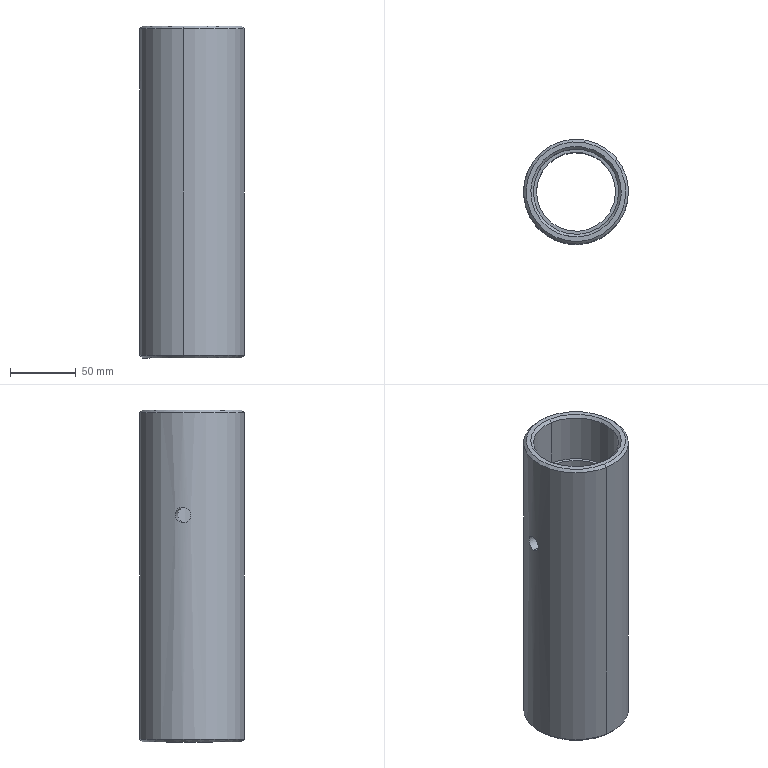Component | SolidWorks | VerticalShaftSleeve-2 | 1 solid | 19 faces | box 80 x 80 x 253 mm | volume 529804 mm3 | cone 8 | cylinder 8 | plane 3 | commonest cylinder face diameters 12 x2 65 x2 80 x2 60.2 x2 | material Q235
build123d program:
from build123d import *

# Parameters (mm, degrees)
SKETCH1_R           = 40
SKETCH1_R_2         = 30.1
BOSS_EXTRUDE1_DEPTH = 253
SKETCH2_R           = 32.5
CUT_EXTRUDE1_DEPTH  = 40
SKETCH3_R           = 6
CUT_EXTRUDE2_DEPTH  = 40
CHAMFER1_SIZE       = 2
CHAMFER2_SIZE       = 2


with BuildPart() as part:
    # Sketch1 → Boss-Extrude1 (new body)
    with BuildSketch(Plane.XY):
        Circle(SKETCH1_R)
        Circle(SKETCH1_R_2, mode=Mode.SUBTRACT)
    extrude(amount=BOSS_EXTRUDE1_DEPTH)

    # Sketch2 → Cut-Extrude1 (cut)
    with BuildSketch(Plane(origin=(0, 0, 0), x_dir=(-1, 0, 0), z_dir=(0, 0, -1))):
        Circle(SKETCH2_R)
    extrude(amount=-CUT_EXTRUDE1_DEPTH, mode=Mode.SUBTRACT)

    # Sketch3 → Cut-Extrude2 (cut)
    with BuildSketch(Plane(origin=(0, 0, 0), x_dir=(1, 0, 0), z_dir=(0, 1, 0))):
        with Locations(Location((0, -80, 0), (0, 0, 270))):
            Circle(SKETCH3_R)
    extrude(amount=-CUT_EXTRUDE2_DEPTH, mode=Mode.SUBTRACT)

    # Chamfer1
    chamfer1_edges = [part.edges().sort_by_distance(p)[0] for p in [
        (-40, 0, 0),
        (-40, 0, 253),
    ]]
    chamfer(chamfer1_edges, length=CHAMFER1_SIZE)

    # Chamfer2
    chamfer2_edges = [part.edges().sort_by_distance(p)[0] for p in [
        (32.5, 0, 0),
        (-30.1, 0, 253),
    ]]
    chamfer(chamfer2_edges, length=CHAMFER2_SIZE)


solid = part.part

# Placed as in the assembly
solid = solid.moved(Location((-277.654, 1601.474, 2931.295), (-180, 0, -80.097)))
STEP:
#1=COLOUR_RGB('',0.7922,0.8196,0.9333);
#2=FILL_AREA_STYLE_COLOUR('',#1);
#3=FILL_AREA_STYLE('',(#2));
#4=SURFACE_STYLE_FILL_AREA(#3);
#5=SURFACE_SIDE_STYLE('',(#4));
#6=SURFACE_STYLE_USAGE(.BOTH.,#5);
#7=PRESENTATION_STYLE_ASSIGNMENT((#6));
#8=CARTESIAN_POINT('',(-10.712,64.311,115.327));
#9=VERTEX_POINT('',#8);
#10=CARTESIAN_POINT('',(-11.151,61.79,115.327));
#11=VERTEX_POINT('',#10);
#12=CARTESIAN_POINT('',(-10.931,63.05,115.327));
#13=DIRECTION('',(-0.,-0.,1.));
#14=DIRECTION('',(0.1718,0.9851,0.));
#15=AXIS2_PLACEMENT_3D('',#12,#13,#14);
#16=CIRCLE('',#15,1.28);
#17=EDGE_CURVE('',#9,#11,#16,.T.);
#18=ORIENTED_EDGE('',*,*,#17,.F.);
#19=CARTESIAN_POINT('',(-10.698,64.388,115.405));
#20=VERTEX_POINT('',#19);
#21=CARTESIAN_POINT('',(-10.712,64.311,115.327));
#22=DIRECTION('',(0.1214,0.6966,0.7071));
#23=VECTOR('',#22,39.37);
#24=LINE('',#21,#23);
#25=EDGE_CURVE('',#9,#20,#24,.T.);
#26=ORIENTED_EDGE('',*,*,#25,.T.);
#27=CARTESIAN_POINT('',(-11.165,61.712,115.405));
#28=VERTEX_POINT('',#27);
#29=CARTESIAN_POINT('',(-10.931,63.05,115.405));
#30=DIRECTION('',(0.,0.,-1.));
#31=DIRECTION('',(0.1718,0.9851,0.));
#32=AXIS2_PLACEMENT_3D('',#29,#30,#31);
#33=CIRCLE('',#32,1.358);
#34=EDGE_CURVE('',#28,#20,#33,.T.);
#35=ORIENTED_EDGE('',*,*,#34,.F.);
#36=CARTESIAN_POINT('',(-11.151,61.79,115.327));
#37=DIRECTION('',(-0.1214,-0.6966,0.7071));
#38=VECTOR('',#37,39.37);
#39=LINE('',#36,#38);
#40=EDGE_CURVE('',#11,#28,#39,.T.);
#41=ORIENTED_EDGE('',*,*,#40,.F.);
#42=EDGE_LOOP('',(#18,#26,#35,#41));
#43=FACE_OUTER_BOUND('',#42,.T.);
#44=CARTESIAN_POINT('',(-10.931,63.05,115.327));
#45=DIRECTION('',(-0.,-0.,1.));
#46=DIRECTION('',(-0.1718,-0.9851,0.));
#47=AXIS2_PLACEMENT_3D('',#44,#45,#46);
#48=CONICAL_SURFACE('',#47,1.28,0.7854);
#49=ADVANCED_FACE('',(#43),#48,.F.);
#50=CARTESIAN_POINT('',(-11.135,61.883,105.523));
#51=VERTEX_POINT('',#50);
#52=CARTESIAN_POINT('',(-10.728,64.218,105.523));
#53=VERTEX_POINT('',#52);
#54=CARTESIAN_POINT('',(-10.931,63.05,105.523));
#55=DIRECTION('',(0.,0.,-1.));
#56=DIRECTION('',(0.1718,0.9851,0.));
#57=AXIS2_PLACEMENT_3D('',#54,#55,#56);
#58=CIRCLE('',#57,1.185);
#59=EDGE_CURVE('',#51,#53,#58,.T.);
#60=ORIENTED_EDGE('',*,*,#59,.F.);
#61=CARTESIAN_POINT('',(-11.148,61.805,105.445));
#62=VERTEX_POINT('',#61);
#63=CARTESIAN_POINT('',(-11.135,61.883,105.523));
#64=DIRECTION('',(-0.1214,-0.6966,-0.7071));
#65=VECTOR('',#64,39.37);
#66=LINE('',#63,#65);
#67=EDGE_CURVE('',#51,#62,#66,.T.);
#68=ORIENTED_EDGE('',*,*,#67,.T.);
#69=CARTESIAN_POINT('',(-10.714,64.295,105.445));
#70=VERTEX_POINT('',#69);
#71=CARTESIAN_POINT('',(-10.931,63.05,105.445));
#72=DIRECTION('',(-0.,-0.,1.));
#73=DIRECTION('',(0.1718,0.9851,0.));
#74=AXIS2_PLACEMENT_3D('',#71,#72,#73);
#75=CIRCLE('',#74,1.264);
#76=EDGE_CURVE('',#70,#62,#75,.T.);
#77=ORIENTED_EDGE('',*,*,#76,.F.);
#78=CARTESIAN_POINT('',(-10.728,64.218,105.523));
#79=DIRECTION('',(0.1214,0.6966,-0.7071));
#80=VECTOR('',#79,39.37);
#81=LINE('',#78,#80);
#82=EDGE_CURVE('',#53,#70,#81,.T.);
#83=ORIENTED_EDGE('',*,*,#82,.F.);
#84=EDGE_LOOP('',(#60,#68,#77,#83));
#85=FACE_OUTER_BOUND('',#84,.T.);
#86=CARTESIAN_POINT('',(-10.931,63.05,105.523));
#87=DIRECTION('',(0.,0.,-1.));
#88=DIRECTION('',(0.1718,0.9851,0.));
#89=AXIS2_PLACEMENT_3D('',#86,#87,#88);
#90=CONICAL_SURFACE('',#89,1.185,0.7854);
#91=ADVANCED_FACE('',(#85),#90,.F.);
#92=CARTESIAN_POINT('',(-11.188,61.576,115.405));
#93=VERTEX_POINT('',#92);
#94=CARTESIAN_POINT('',(-10.674,64.524,115.405));
#95=VERTEX_POINT('',#94);
#96=CARTESIAN_POINT('',(-10.931,63.05,115.405));
#97=DIRECTION('',(-0.,-0.,1.));
#98=DIRECTION('',(0.1718,0.9851,0.));
#99=AXIS2_PLACEMENT_3D('',#96,#97,#98);
#100=CIRCLE('',#99,1.496);
#101=EDGE_CURVE('',#93,#95,#100,.T.);
#102=ORIENTED_EDGE('',*,*,#101,.F.);
#103=CARTESIAN_POINT('',(-11.202,61.499,115.327));
#104=VERTEX_POINT('',#103);
#105=CARTESIAN_POINT('',(-11.202,61.499,115.327));
#106=DIRECTION('',(-0.1214,-0.6966,-0.7071));
#107=VECTOR('',#106,39.37);
#108=LINE('',#105,#107);
#109=EDGE_CURVE('',#93,#104,#108,.T.);
#110=ORIENTED_EDGE('',*,*,#109,.T.);
#111=CARTESIAN_POINT('',(-10.661,64.602,115.327));
#112=VERTEX_POINT('',#111);
#113=CARTESIAN_POINT('',(-10.931,63.05,115.327));
#114=DIRECTION('',(0.,0.,-1.));
#115=DIRECTION('',(0.1718,0.9851,0.));
#116=AXIS2_PLACEMENT_3D('',#113,#114,#115);
#117=CIRCLE('',#116,1.575);
#118=EDGE_CURVE('',#112,#104,#117,.T.);
#119=ORIENTED_EDGE('',*,*,#118,.F.);
#120=CARTESIAN_POINT('',(-10.661,64.602,115.327));
#121=DIRECTION('',(0.1214,0.6966,-0.7071));
#122=VECTOR('',#121,39.37);
#123=LINE('',#120,#122);
#124=EDGE_CURVE('',#95,#112,#123,.T.);
#125=ORIENTED_EDGE('',*,*,#124,.F.);
#126=EDGE_LOOP('',(#102,#110,#119,#125));
#127=FACE_OUTER_BOUND('',#126,.T.);
#128=CARTESIAN_POINT('',(-10.931,63.05,115.327));
#129=DIRECTION('',(0.,0.,-1.));
#130=DIRECTION('',(0.1718,0.9851,0.));
#131=AXIS2_PLACEMENT_3D('',#128,#129,#130);
#132=CONICAL_SURFACE('',#131,1.575,0.7854);
#133=ADVANCED_FACE('',(#127),#132,.T.);
#134=CARTESIAN_POINT('',(-10.674,64.524,105.445));
#135=VERTEX_POINT('',#134);
#136=CARTESIAN_POINT('',(-11.188,61.576,105.445));
#137=VERTEX_POINT('',#136);
#138=CARTESIAN_POINT('',(-10.931,63.05,105.445));
#139=DIRECTION('',(0.,0.,-1.));
#140=DIRECTION('',(0.1718,0.9851,0.));
#141=AXIS2_PLACEMENT_3D('',#138,#139,#140);
#142=CIRCLE('',#141,1.496);
#143=EDGE_CURVE('',#135,#137,#142,.T.);
#144=ORIENTED_EDGE('',*,*,#143,.F.);
#145=CARTESIAN_POINT('',(-10.661,64.602,105.523));
#146=VERTEX_POINT('',#145);
#147=CARTESIAN_POINT('',(-10.674,64.524,105.445));
#148=DIRECTION('',(0.1214,0.6966,0.7071));
#149=VECTOR('',#148,39.37);
#150=LINE('',#147,#149);
#151=EDGE_CURVE('',#135,#146,#150,.T.);
#152=ORIENTED_EDGE('',*,*,#151,.T.);
#153=CARTESIAN_POINT('',(-11.202,61.499,105.523));
#154=VERTEX_POINT('',#153);
#155=CARTESIAN_POINT('',(-10.931,63.05,105.523));
#156=DIRECTION('',(-0.,-0.,1.));
#157=DIRECTION('',(0.1718,0.9851,0.));
#158=AXIS2_PLACEMENT_3D('',#155,#156,#157);
#159=CIRCLE('',#158,1.575);
#160=EDGE_CURVE('',#154,#146,#159,.T.);
#161=ORIENTED_EDGE('',*,*,#160,.F.);
#162=CARTESIAN_POINT('',(-11.188,61.576,105.445));
#163=DIRECTION('',(-0.1214,-0.6966,0.7071));
#164=VECTOR('',#163,39.37);
#165=LINE('',#162,#164);
#166=EDGE_CURVE('',#137,#154,#165,.T.);
#167=ORIENTED_EDGE('',*,*,#166,.F.);
#168=EDGE_LOOP('',(#144,#152,#161,#167));
#169=FACE_OUTER_BOUND('',#168,.T.);
#170=CARTESIAN_POINT('',(-10.931,63.05,105.445));
#171=DIRECTION('',(-0.,-0.,1.));
#172=DIRECTION('',(-0.1718,-0.9851,0.));
#173=AXIS2_PLACEMENT_3D('',#170,#171,#172);
#174=CONICAL_SURFACE('',#173,1.496,0.7854);
#175=ADVANCED_FACE('',(#169),#174,.T.);
#176=CARTESIAN_POINT('',(-12.483,63.321,112.492));
#177=VERTEX_POINT('',#176);
#178=CARTESIAN_POINT('',(-12.483,63.321,112.019));
#179=VERTEX_POINT('',#178);
#180=CARTESIAN_POINT('',(-12.483,63.321,112.492));
#181=CARTESIAN_POINT('',(-12.485,63.305,112.492));
#182=CARTESIAN_POINT('',(-12.488,63.29,112.49));
#183=CARTESIAN_POINT('',(-12.492,63.26,112.484));
#184=CARTESIAN_POINT('',(-12.494,63.245,112.48));
#185=CARTESIAN_POINT('',(-12.496,63.224,112.471));
#186=CARTESIAN_POINT('',(-12.497,63.217,112.468));
#187=CARTESIAN_POINT('',(-12.499,63.204,112.46));
#188=CARTESIAN_POINT('',(-12.499,63.197,112.456));
#189=CARTESIAN_POINT('',(-12.501,63.177,112.443));
#190=CARTESIAN_POINT('',(-12.502,63.166,112.434));
#191=CARTESIAN_POINT('',(-12.503,63.144,112.412));
#192=CARTESIAN_POINT('',(-12.504,63.134,112.4));
#193=CARTESIAN_POINT('',(-12.505,63.116,112.374));
#194=CARTESIAN_POINT('',(-12.505,63.109,112.361));
#195=CARTESIAN_POINT('',(-12.505,63.1,112.339));
#196=CARTESIAN_POINT('',(-12.505,63.097,112.332));
#197=CARTESIAN_POINT('',(-12.505,63.093,112.317));
#198=CARTESIAN_POINT('',(-12.506,63.091,112.31));
#199=CARTESIAN_POINT('',(-12.506,63.086,112.287));
#200=CARTESIAN_POINT('',(-12.506,63.085,112.271));
#201=CARTESIAN_POINT('',(-12.506,63.085,112.24));
#202=CARTESIAN_POINT('',(-12.506,63.086,112.225));
#203=CARTESIAN_POINT('',(-12.506,63.091,112.202));
#204=CARTESIAN_POINT('',(-12.505,63.093,112.195));
#205=CARTESIAN_POINT('',(-12.505,63.097,112.18));
#206=CARTESIAN_POINT('',(-12.505,63.1,112.172));
#207=CARTESIAN_POINT('',(-12.505,63.109,112.151));
#208=CARTESIAN_POINT('',(-12.505,63.116,112.137));
#209=CARTESIAN_POINT('',(-12.504,63.134,112.112));
#210=CARTESIAN_POINT('',(-12.503,63.144,112.1));
#211=CARTESIAN_POINT('',(-12.502,63.165,112.078));
#212=CARTESIAN_POINT('',(-12.501,63.177,112.068));
#213=CARTESIAN_POINT('',(-12.499,63.203,112.051));
#214=CARTESIAN_POINT('',(-12.497,63.217,112.044));
#215=CARTESIAN_POINT('',(-12.495,63.238,112.035));
#216=CARTESIAN_POINT('',(-12.494,63.245,112.032));
#217=CARTESIAN_POINT('',(-12.492,63.26,112.028));
#218=CARTESIAN_POINT('',(-12.491,63.267,112.026));
#219=CARTESIAN_POINT('',(-12.488,63.29,112.021));
#220=CARTESIAN_POINT('',(-12.485,63.305,112.019));
#221=CARTESIAN_POINT('',(-12.483,63.321,112.019));
#222=B_SPLINE_CURVE_WITH_KNOTS('',3,(#180,#181,#182,#183,#184,#185,#186,#187,#188,#189,#190,#191,#192,#193,#194,#195,#196,#197,#198,#199,#200,#201,#202,#203,#204,#205,#206,#207,#208,#209,#210,#211,#212,#213,#214,#215,#216,#217,#218,#219,#220,#221),.UNSPECIFIED.,.F.,.F.,(4,2,2,2,2,2,2,2,2,2,2,2,2,2,2,2,2,2,2,2,4),(0.01879,0.01996,0.02113,0.02172,0.02231,0.02348,0.02465,0.02583,0.02641,0.027,0.02818,0.02935,0.02994,0.03052,0.0317,0.03287,0.03404,0.03522,0.03581,0.03639,0.03757),.UNSPECIFIED.);
#223=EDGE_CURVE('',#177,#179,#222,.T.);
#224=ORIENTED_EDGE('',*,*,#223,.F.);
#225=CARTESIAN_POINT('',(-12.099,63.254,112.492));
#226=VERTEX_POINT('',#225);
#227=CARTESIAN_POINT('',(-12.483,63.321,112.492));
#228=DIRECTION('',(0.9851,-0.1718,0.));
#229=VECTOR('',#228,39.37);
#230=LINE('',#227,#229);
#231=EDGE_CURVE('',#177,#226,#230,.T.);
#232=ORIENTED_EDGE('',*,*,#231,.T.);
#233=CARTESIAN_POINT('',(-12.099,63.254,112.019));
#234=VERTEX_POINT('',#233);
#235=CARTESIAN_POINT('',(-12.099,63.254,112.492));
#236=CARTESIAN_POINT('',(-12.101,63.238,112.492));
#237=CARTESIAN_POINT('',(-12.104,63.223,112.49));
#238=CARTESIAN_POINT('',(-12.108,63.193,112.484));
#239=CARTESIAN_POINT('',(-12.109,63.178,112.48));
#240=CARTESIAN_POINT('',(-12.112,63.157,112.471));
#241=CARTESIAN_POINT('',(-12.112,63.15,112.468));
#242=CARTESIAN_POINT('',(-12.113,63.136,112.46));
#243=CARTESIAN_POINT('',(-12.114,63.13,112.456));
#244=CARTESIAN_POINT('',(-12.115,63.11,112.443));
#245=CARTESIAN_POINT('',(-12.115,63.098,112.434));
#246=CARTESIAN_POINT('',(-12.116,63.076,112.412));
#247=CARTESIAN_POINT('',(-12.116,63.066,112.4));
#248=CARTESIAN_POINT('',(-12.116,63.049,112.374));
#249=CARTESIAN_POINT('',(-12.116,63.041,112.361));
#250=CARTESIAN_POINT('',(-12.116,63.032,112.339));
#251=CARTESIAN_POINT('',(-12.116,63.03,112.332));
#252=CARTESIAN_POINT('',(-12.116,63.025,112.317));
#253=CARTESIAN_POINT('',(-12.116,63.023,112.31));
#254=CARTESIAN_POINT('',(-12.116,63.018,112.287));
#255=CARTESIAN_POINT('',(-12.116,63.017,112.271));
#256=CARTESIAN_POINT('',(-12.116,63.017,112.24));
#257=CARTESIAN_POINT('',(-12.116,63.018,112.225));
#258=CARTESIAN_POINT('',(-12.116,63.025,112.195));
#259=CARTESIAN_POINT('',(-12.116,63.029,112.18));
#260=CARTESIAN_POINT('',(-12.116,63.041,112.151));
#261=CARTESIAN_POINT('',(-12.116,63.049,112.137));
#262=CARTESIAN_POINT('',(-12.116,63.062,112.118));
#263=CARTESIAN_POINT('',(-12.116,63.066,112.112));
#264=CARTESIAN_POINT('',(-12.116,63.076,112.1));
#265=CARTESIAN_POINT('',(-12.116,63.082,112.094));
#266=CARTESIAN_POINT('',(-12.115,63.098,112.078));
#267=CARTESIAN_POINT('',(-12.115,63.11,112.068));
#268=CARTESIAN_POINT('',(-12.113,63.136,112.051));
#269=CARTESIAN_POINT('',(-12.112,63.15,112.044));
#270=CARTESIAN_POINT('',(-12.11,63.171,112.035));
#271=CARTESIAN_POINT('',(-12.109,63.178,112.032));
#272=CARTESIAN_POINT('',(-12.108,63.193,112.028));
#273=CARTESIAN_POINT('',(-12.107,63.2,112.026));
#274=CARTESIAN_POINT('',(-12.104,63.223,112.021));
#275=CARTESIAN_POINT('',(-12.101,63.238,112.019));
#276=CARTESIAN_POINT('',(-12.099,63.254,112.019));
#277=B_SPLINE_CURVE_WITH_KNOTS('',3,(#235,#236,#237,#238,#239,#240,#241,#242,#243,#244,#245,#246,#247,#248,#249,#250,#251,#252,#253,#254,#255,#256,#257,#258,#259,#260,#261,#262,#263,#264,#265,#266,#267,#268,#269,#270,#271,#272,#273,#274,#275,#276),.UNSPECIFIED.,.F.,.F.,(4,2,2,2,2,2,2,2,2,2,2,2,2,2,2,2,2,2,2,2,4),(0.01881,0.01998,0.02116,0.02174,0.02233,0.02351,0.02468,0.02586,0.02644,0.02703,0.02821,0.02938,0.03056,0.03173,0.03232,0.03291,0.03408,0.03526,0.03584,0.03643,0.03761),.UNSPECIFIED.);
#278=EDGE_CURVE('',#226,#234,#277,.T.);
#279=ORIENTED_EDGE('',*,*,#278,.T.);
#280=CARTESIAN_POINT('',(-12.483,63.321,112.019));
#281=DIRECTION('',(0.9851,-0.1718,0.));
#282=VECTOR('',#281,39.37);
#283=LINE('',#280,#282);
#284=EDGE_CURVE('',#179,#234,#283,.T.);
#285=ORIENTED_EDGE('',*,*,#284,.F.);
#286=EDGE_LOOP('',(#224,#232,#279,#285));
#287=FACE_OUTER_BOUND('',#286,.T.);
#288=CARTESIAN_POINT('',(-12.483,63.321,112.256));
#289=DIRECTION('',(0.9851,-0.1718,0.));
#290=DIRECTION('',(0.,0.,-1.));
#291=AXIS2_PLACEMENT_3D('',#288,#289,#290);
#292=CYLINDRICAL_SURFACE('',#291,0.2362);
#293=ADVANCED_FACE('',(#287),#292,.F.);
#294=CARTESIAN_POINT('',(-10.712,64.311,113.831));
#295=VERTEX_POINT('',#294);
#296=CARTESIAN_POINT('',(-11.151,61.79,113.831));
#297=VERTEX_POINT('',#296);
#298=CARTESIAN_POINT('',(-10.931,63.05,113.831));
#299=DIRECTION('',(-0.,-0.,1.));
#300=DIRECTION('',(-0.1718,-0.9851,0.));
#301=AXIS2_PLACEMENT_3D('',#298,#299,#300);
#302=CIRCLE('',#301,1.28);
#303=EDGE_CURVE('',#295,#297,#302,.T.);
#304=ORIENTED_EDGE('',*,*,#303,.F.);
#305=CARTESIAN_POINT('',(-10.712,64.311,113.831));
#306=DIRECTION('',(-0.,-0.,1.));
#307=VECTOR('',#306,39.37);
#308=LINE('',#305,#307);
#309=EDGE_CURVE('',#295,#9,#308,.T.);
#310=ORIENTED_EDGE('',*,*,#309,.T.);
#311=ORIENTED_EDGE('',*,*,#17,.T.);
#312=CARTESIAN_POINT('',(-11.151,61.79,113.831));
#313=DIRECTION('',(-0.,-0.,1.));
#314=VECTOR('',#313,39.37);
#315=LINE('',#312,#314);
#316=EDGE_CURVE('',#297,#11,#315,.T.);
#317=ORIENTED_EDGE('',*,*,#316,.F.);
#318=EDGE_LOOP('',(#304,#310,#311,#317));
#319=FACE_OUTER_BOUND('',#318,.T.);
#320=CARTESIAN_POINT('',(-10.931,63.05,113.831));
#321=DIRECTION('',(-0.,-0.,1.));
#322=DIRECTION('',(-0.1718,-0.9851,0.));
#323=AXIS2_PLACEMENT_3D('',#320,#321,#322);
#324=CYLINDRICAL_SURFACE('',#323,1.28);
#325=ADVANCED_FACE('',(#319),#324,.F.);
#326=ORIENTED_EDGE('',*,*,#160,.T.);
#327=CARTESIAN_POINT('',(-10.661,64.602,105.445));
#328=DIRECTION('',(-0.,-0.,1.));
#329=VECTOR('',#328,39.37);
#330=LINE('',#327,#329);
#331=EDGE_CURVE('',#146,#112,#330,.T.);
#332=ORIENTED_EDGE('',*,*,#331,.T.);
#333=ORIENTED_EDGE('',*,*,#118,.T.);
#334=CARTESIAN_POINT('',(-11.202,61.499,105.445));
#335=DIRECTION('',(-0.,-0.,1.));
#336=VECTOR('',#335,39.37);
#337=LINE('',#334,#336);
#338=EDGE_CURVE('',#154,#104,#337,.T.);
#339=ORIENTED_EDGE('',*,*,#338,.F.);
#340=EDGE_LOOP('',(#326,#332,#333,#339));
#341=FACE_OUTER_BOUND('',#340,.T.);
#342=CARTESIAN_POINT('',(-10.931,63.05,105.445));
#343=DIRECTION('',(-0.,-0.,1.));
#344=DIRECTION('',(-0.1718,-0.9851,0.));
#345=AXIS2_PLACEMENT_3D('',#342,#343,#344);
#346=CYLINDRICAL_SURFACE('',#345,1.575);
#347=ADVANCED_FACE('',(#341),#346,.T.);
#348=CARTESIAN_POINT('',(-12.099,63.254,112.019));
#349=CARTESIAN_POINT('',(-12.096,63.269,112.019));
#350=CARTESIAN_POINT('',(-12.093,63.284,112.021));
#351=CARTESIAN_POINT('',(-12.088,63.306,112.026));
#352=CARTESIAN_POINT('',(-12.087,63.314,112.027));
#353=CARTESIAN_POINT('',(-12.083,63.328,112.032));
#354=CARTESIAN_POINT('',(-12.081,63.335,112.035));
#355=CARTESIAN_POINT('',(-12.076,63.356,112.043));
#356=CARTESIAN_POINT('',(-12.073,63.369,112.051));
#357=CARTESIAN_POINT('',(-12.065,63.394,112.068));
#358=CARTESIAN_POINT('',(-12.062,63.406,112.078));
#359=CARTESIAN_POINT('',(-12.055,63.427,112.1));
#360=CARTESIAN_POINT('',(-12.052,63.436,112.111));
#361=CARTESIAN_POINT('',(-12.046,63.453,112.137));
#362=CARTESIAN_POINT('',(-12.043,63.46,112.151));
#363=CARTESIAN_POINT('',(-12.04,63.468,112.172));
#364=CARTESIAN_POINT('',(-12.039,63.47,112.18));
#365=CARTESIAN_POINT('',(-12.038,63.475,112.194));
#366=CARTESIAN_POINT('',(-12.037,63.477,112.202));
#367=CARTESIAN_POINT('',(-12.035,63.481,112.225));
#368=CARTESIAN_POINT('',(-12.035,63.482,112.24));
#369=CARTESIAN_POINT('',(-12.035,63.482,112.271));
#370=CARTESIAN_POINT('',(-12.035,63.481,112.287));
#371=CARTESIAN_POINT('',(-12.038,63.475,112.317));
#372=CARTESIAN_POINT('',(-12.039,63.471,112.332));
#373=CARTESIAN_POINT('',(-12.042,63.462,112.353));
#374=CARTESIAN_POINT('',(-12.043,63.459,112.36));
#375=CARTESIAN_POINT('',(-12.046,63.452,112.374));
#376=CARTESIAN_POINT('',(-12.047,63.448,112.381));
#377=CARTESIAN_POINT('',(-12.052,63.436,112.4));
#378=CARTESIAN_POINT('',(-12.055,63.427,112.412));
#379=CARTESIAN_POINT('',(-12.062,63.406,112.434));
#380=CARTESIAN_POINT('',(-12.065,63.394,112.443));
#381=CARTESIAN_POINT('',(-12.071,63.376,112.456));
#382=CARTESIAN_POINT('',(-12.073,63.369,112.46));
#383=CARTESIAN_POINT('',(-12.076,63.356,112.468));
#384=CARTESIAN_POINT('',(-12.078,63.349,112.471));
#385=CARTESIAN_POINT('',(-12.083,63.328,112.48));
#386=CARTESIAN_POINT('',(-12.087,63.314,112.484));
#387=CARTESIAN_POINT('',(-12.091,63.292,112.489));
#388=CARTESIAN_POINT('',(-12.093,63.284,112.49));
#389=CARTESIAN_POINT('',(-12.096,63.269,112.492));
#390=CARTESIAN_POINT('',(-12.097,63.261,112.492));
#391=CARTESIAN_POINT('',(-12.099,63.254,112.492));
#392=B_SPLINE_CURVE_WITH_KNOTS('',3,(#348,#349,#350,#351,#352,#353,#354,#355,#356,#357,#358,#359,#360,#361,#362,#363,#364,#365,#366,#367,#368,#369,#370,#371,#372,#373,#374,#375,#376,#377,#378,#379,#380,#381,#382,#383,#384,#385,#386,#387,#388,#389,#390,#391),.UNSPECIFIED.,.F.,.F.,(4,2,2,2,2,2,2,2,2,2,2,2,2,2,2,2,2,2,2,2,2,4),(0.,0.001175,0.001763,0.002351,0.003526,0.004701,0.005877,0.007052,0.00764,0.008228,0.009403,0.01058,0.01175,0.01234,0.01293,0.0141,0.01528,0.01587,0.01646,0.01763,0.01822,0.01881),.UNSPECIFIED.);
#393=EDGE_CURVE('',#234,#226,#392,.T.);
#394=ORIENTED_EDGE('',*,*,#393,.F.);
#395=ORIENTED_EDGE('',*,*,#278,.F.);
#396=EDGE_LOOP('',(#394,#395));
#397=FACE_BOUND('',#396,.T.);
#398=ORIENTED_EDGE('',*,*,#59,.T.);
#399=CARTESIAN_POINT('',(-10.728,64.218,113.831));
#400=VERTEX_POINT('',#399);
#401=CARTESIAN_POINT('',(-10.728,64.218,105.445));
#402=DIRECTION('',(-0.,-0.,1.));
#403=VECTOR('',#402,39.37);
#404=LINE('',#401,#403);
#405=EDGE_CURVE('',#53,#400,#404,.T.);
#406=ORIENTED_EDGE('',*,*,#405,.T.);
#407=CARTESIAN_POINT('',(-11.135,61.883,113.831));
#408=VERTEX_POINT('',#407);
#409=CARTESIAN_POINT('',(-10.931,63.05,113.831));
#410=DIRECTION('',(-0.,-0.,1.));
#411=DIRECTION('',(-0.1718,-0.9851,0.));
#412=AXIS2_PLACEMENT_3D('',#409,#410,#411);
#413=CIRCLE('',#412,1.185);
#414=EDGE_CURVE('',#400,#408,#413,.T.);
#415=ORIENTED_EDGE('',*,*,#414,.T.);
#416=CARTESIAN_POINT('',(-11.135,61.883,105.445));
#417=DIRECTION('',(-0.,-0.,1.));
#418=VECTOR('',#417,39.37);
#419=LINE('',#416,#418);
#420=EDGE_CURVE('',#51,#408,#419,.T.);
#421=ORIENTED_EDGE('',*,*,#420,.F.);
#422=EDGE_LOOP('',(#398,#406,#415,#421));
#423=FACE_OUTER_BOUND('',#422,.T.);
#424=CARTESIAN_POINT('',(-10.931,63.05,105.445));
#425=DIRECTION('',(-0.,-0.,1.));
#426=DIRECTION('',(-0.1718,-0.9851,0.));
#427=AXIS2_PLACEMENT_3D('',#424,#425,#426);
#428=CYLINDRICAL_SURFACE('',#427,1.185);
#429=ADVANCED_FACE('',(#397,#423),#428,.F.);
#430=ORIENTED_EDGE('',*,*,#405,.F.);
#431=CARTESIAN_POINT('',(-10.931,63.05,105.523));
#432=DIRECTION('',(0.,0.,-1.));
#433=DIRECTION('',(0.1718,0.9851,0.));
#434=AXIS2_PLACEMENT_3D('',#431,#432,#433);
#435=CIRCLE('',#434,1.185);
#436=EDGE_CURVE('',#53,#51,#435,.T.);
#437=ORIENTED_EDGE('',*,*,#436,.T.);
#438=ORIENTED_EDGE('',*,*,#420,.T.);
#439=CARTESIAN_POINT('',(-10.931,63.05,113.831));
#440=DIRECTION('',(-0.,-0.,1.));
#441=DIRECTION('',(-0.1718,-0.9851,0.));
#442=AXIS2_PLACEMENT_3D('',#439,#440,#441);
#443=CIRCLE('',#442,1.185);
#444=EDGE_CURVE('',#408,#400,#443,.T.);
#445=ORIENTED_EDGE('',*,*,#444,.T.);
#446=EDGE_LOOP('',(#430,#437,#438,#445));
#447=FACE_OUTER_BOUND('',#446,.T.);
#448=CARTESIAN_POINT('',(-10.931,63.05,105.445));
#449=DIRECTION('',(-0.,-0.,1.));
#450=DIRECTION('',(-0.1718,-0.9851,0.));
#451=AXIS2_PLACEMENT_3D('',#448,#449,#450);
#452=CYLINDRICAL_SURFACE('',#451,1.185);
#453=ADVANCED_FACE('',(#447),#452,.F.);
#454=ORIENTED_EDGE('',*,*,#76,.T.);
#455=CARTESIAN_POINT('',(-10.931,63.05,105.445));
#456=DIRECTION('',(-0.,-0.,1.));
#457=DIRECTION('',(0.1718,0.9851,0.));
#458=AXIS2_PLACEMENT_3D('',#455,#456,#457);
#459=CIRCLE('',#458,1.264);
#460=EDGE_CURVE('',#62,#70,#459,.T.);
#461=ORIENTED_EDGE('',*,*,#460,.T.);
#462=EDGE_LOOP('',(#454,#461));
#463=FACE_BOUND('',#462,.T.);
#464=CARTESIAN_POINT('',(-10.931,63.05,105.445));
#465=DIRECTION('',(0.,0.,-1.));
#466=DIRECTION('',(0.1718,0.9851,0.));
#467=AXIS2_PLACEMENT_3D('',#464,#465,#466);
#468=CIRCLE('',#467,1.496);
#469=EDGE_CURVE('',#137,#135,#468,.T.);
#470=ORIENTED_EDGE('',*,*,#469,.T.);
#471=ORIENTED_EDGE('',*,*,#143,.T.);
#472=EDGE_LOOP('',(#470,#471));
#473=FACE_OUTER_BOUND('',#472,.T.);
#474=CARTESIAN_POINT('',(-10.931,63.05,105.445));
#475=DIRECTION('',(0.,0.,-1.));
#476=DIRECTION('',(0.1718,0.9851,0.));
#477=AXIS2_PLACEMENT_3D('',#474,#475,#476);
#478=PLANE('',#477);
#479=ADVANCED_FACE('',(#463,#473),#478,.T.);
#480=ORIENTED_EDGE('',*,*,#34,.T.);
#481=CARTESIAN_POINT('',(-10.931,63.05,115.405));
#482=DIRECTION('',(0.,0.,-1.));
#483=DIRECTION('',(0.1718,0.9851,0.));
#484=AXIS2_PLACEMENT_3D('',#481,#482,#483);
#485=CIRCLE('',#484,1.358);
#486=EDGE_CURVE('',#20,#28,#485,.T.);
#487=ORIENTED_EDGE('',*,*,#486,.T.);
#488=EDGE_LOOP('',(#480,#487));
#489=FACE_BOUND('',#488,.T.);
#490=CARTESIAN_POINT('',(-10.931,63.05,115.405));
#491=DIRECTION('',(-0.,-0.,1.));
#492=DIRECTION('',(0.1718,0.9851,0.));
#493=AXIS2_PLACEMENT_3D('',#490,#491,#492);
#494=CIRCLE('',#493,1.496);
#495=EDGE_CURVE('',#95,#93,#494,.T.);
#496=ORIENTED_EDGE('',*,*,#495,.T.);
#497=ORIENTED_EDGE('',*,*,#101,.T.);
#498=EDGE_LOOP('',(#496,#497));
#499=FACE_OUTER_BOUND('',#498,.T.);
#500=CARTESIAN_POINT('',(-10.931,63.05,115.405));
#501=DIRECTION('',(0.,0.,-1.));
#502=DIRECTION('',(0.1718,0.9851,0.));
#503=AXIS2_PLACEMENT_3D('',#500,#501,#502);
#504=PLANE('',#503);
#505=ADVANCED_FACE('',(#489,#499),#504,.F.);
#506=ORIENTED_EDGE('',*,*,#331,.F.);
#507=CARTESIAN_POINT('',(-10.931,63.05,105.523));
#508=DIRECTION('',(-0.,-0.,1.));
#509=DIRECTION('',(0.1718,0.9851,0.));
#510=AXIS2_PLACEMENT_3D('',#507,#508,#509);
#511=CIRCLE('',#510,1.575);
#512=EDGE_CURVE('',#146,#154,#511,.T.);
#513=ORIENTED_EDGE('',*,*,#512,.T.);
#514=ORIENTED_EDGE('',*,*,#338,.T.);
#515=CARTESIAN_POINT('',(-10.931,63.05,115.327));
#516=DIRECTION('',(0.,0.,-1.));
#517=DIRECTION('',(0.1718,0.9851,0.));
#518=AXIS2_PLACEMENT_3D('',#515,#516,#517);
#519=CIRCLE('',#518,1.575);
#520=EDGE_CURVE('',#104,#112,#519,.T.);
#521=ORIENTED_EDGE('',*,*,#520,.T.);
#522=EDGE_LOOP('',(#506,#513,#514,#521));
#523=FACE_OUTER_BOUND('',#522,.T.);
#524=CARTESIAN_POINT('',(-12.483,63.321,112.019));
#525=CARTESIAN_POINT('',(-12.48,63.336,112.019));
#526=CARTESIAN_POINT('',(-12.477,63.351,112.021));
#527=CARTESIAN_POINT('',(-12.473,63.373,112.026));
#528=CARTESIAN_POINT('',(-12.471,63.381,112.027));
#529=CARTESIAN_POINT('',(-12.468,63.395,112.032));
#530=CARTESIAN_POINT('',(-12.466,63.402,112.035));
#531=CARTESIAN_POINT('',(-12.461,63.423,112.043));
#532=CARTESIAN_POINT('',(-12.458,63.437,112.051));
#533=CARTESIAN_POINT('',(-12.451,63.461,112.068));
#534=CARTESIAN_POINT('',(-12.448,63.473,112.078));
#535=CARTESIAN_POINT('',(-12.442,63.494,112.1));
#536=CARTESIAN_POINT('',(-12.439,63.504,112.111));
#537=CARTESIAN_POINT('',(-12.436,63.516,112.131));
#538=CARTESIAN_POINT('',(-12.434,63.52,112.138));
#539=CARTESIAN_POINT('',(-12.432,63.527,112.151));
#540=CARTESIAN_POINT('',(-12.43,63.533,112.165));
#541=CARTESIAN_POINT('',(-12.429,63.538,112.18));
#542=CARTESIAN_POINT('',(-12.427,63.543,112.194));
#543=CARTESIAN_POINT('',(-12.426,63.544,112.202));
#544=CARTESIAN_POINT('',(-12.425,63.549,112.225));
#545=CARTESIAN_POINT('',(-12.425,63.55,112.24));
#546=CARTESIAN_POINT('',(-12.425,63.55,112.271));
#547=CARTESIAN_POINT('',(-12.425,63.549,112.287));
#548=CARTESIAN_POINT('',(-12.427,63.543,112.317));
#549=CARTESIAN_POINT('',(-12.428,63.539,112.332));
#550=CARTESIAN_POINT('',(-12.431,63.53,112.353));
#551=CARTESIAN_POINT('',(-12.432,63.527,112.36));
#552=CARTESIAN_POINT('',(-12.434,63.52,112.374));
#553=CARTESIAN_POINT('',(-12.436,63.516,112.381));
#554=CARTESIAN_POINT('',(-12.439,63.504,112.4));
#555=CARTESIAN_POINT('',(-12.442,63.494,112.412));
#556=CARTESIAN_POINT('',(-12.448,63.473,112.434));
#557=CARTESIAN_POINT('',(-12.451,63.461,112.443));
#558=CARTESIAN_POINT('',(-12.456,63.443,112.456));
#559=CARTESIAN_POINT('',(-12.458,63.436,112.46));
#560=CARTESIAN_POINT('',(-12.461,63.423,112.468));
#561=CARTESIAN_POINT('',(-12.463,63.416,112.471));
#562=CARTESIAN_POINT('',(-12.468,63.395,112.48));
#563=CARTESIAN_POINT('',(-12.471,63.381,112.484));
#564=CARTESIAN_POINT('',(-12.477,63.351,112.49));
#565=CARTESIAN_POINT('',(-12.48,63.336,112.492));
#566=CARTESIAN_POINT('',(-12.483,63.321,112.492));
#567=B_SPLINE_CURVE_WITH_KNOTS('',3,(#524,#525,#526,#527,#528,#529,#530,#531,#532,#533,#534,#535,#536,#537,#538,#539,#540,#541,#542,#543,#544,#545,#546,#547,#548,#549,#550,#551,#552,#553,#554,#555,#556,#557,#558,#559,#560,#561,#562,#563,#564,#565,#566),.UNSPECIFIED.,.F.,.F.,(4,2,2,2,2,2,2,2,1,2,2,2,2,2,2,2,2,2,2,2,2,4),(0.,0.001174,0.001761,0.002348,0.003522,0.004696,0.00587,0.006457,0.007044,0.007632,0.008219,0.009393,0.01057,0.01174,0.01233,0.01291,0.01409,0.01526,0.01585,0.01644,0.01761,0.01879),.UNSPECIFIED.);
#568=EDGE_CURVE('',#179,#177,#567,.T.);
#569=ORIENTED_EDGE('',*,*,#568,.T.);
#570=ORIENTED_EDGE('',*,*,#223,.T.);
#571=EDGE_LOOP('',(#569,#570));
#572=FACE_BOUND('',#571,.T.);
#573=CARTESIAN_POINT('',(-10.931,63.05,105.445));
#574=DIRECTION('',(-0.,-0.,1.));
#575=DIRECTION('',(-0.1718,-0.9851,0.));
#576=AXIS2_PLACEMENT_3D('',#573,#574,#575);
#577=CYLINDRICAL_SURFACE('',#576,1.575);
#578=ADVANCED_FACE('',(#523,#572),#577,.T.);
#579=ORIENTED_EDGE('',*,*,#309,.F.);
#580=CARTESIAN_POINT('',(-10.931,63.05,113.831));
#581=DIRECTION('',(-0.,-0.,1.));
#582=DIRECTION('',(-0.1718,-0.9851,0.));
#583=AXIS2_PLACEMENT_3D('',#580,#581,#582);
#584=CIRCLE('',#583,1.28);
#585=EDGE_CURVE('',#297,#295,#584,.T.);
#586=ORIENTED_EDGE('',*,*,#585,.F.);
#587=ORIENTED_EDGE('',*,*,#316,.T.);
#588=CARTESIAN_POINT('',(-10.931,63.05,115.327));
#589=DIRECTION('',(-0.,-0.,1.));
#590=DIRECTION('',(0.1718,0.9851,0.));
#591=AXIS2_PLACEMENT_3D('',#588,#589,#590);
#592=CIRCLE('',#591,1.28);
#593=EDGE_CURVE('',#11,#9,#592,.T.);
#594=ORIENTED_EDGE('',*,*,#593,.T.);
#595=EDGE_LOOP('',(#579,#586,#587,#594));
#596=FACE_OUTER_BOUND('',#595,.T.);
#597=CARTESIAN_POINT('',(-10.931,63.05,113.831));
#598=DIRECTION('',(-0.,-0.,1.));
#599=DIRECTION('',(-0.1718,-0.9851,0.));
#600=AXIS2_PLACEMENT_3D('',#597,#598,#599);
#601=CYLINDRICAL_SURFACE('',#600,1.28);
#602=ADVANCED_FACE('',(#596),#601,.F.);
#603=ORIENTED_EDGE('',*,*,#444,.F.);
#604=ORIENTED_EDGE('',*,*,#414,.F.);
#605=EDGE_LOOP('',(#603,#604));
#606=FACE_BOUND('',#605,.T.);
#607=ORIENTED_EDGE('',*,*,#585,.T.);
#608=ORIENTED_EDGE('',*,*,#303,.T.);
#609=EDGE_LOOP('',(#607,#608));
#610=FACE_OUTER_BOUND('',#609,.T.);
#611=CARTESIAN_POINT('',(-10.931,63.05,113.831));
#612=DIRECTION('',(-0.,-0.,1.));
#613=DIRECTION('',(-0.1718,-0.9851,-0.));
#614=AXIS2_PLACEMENT_3D('',#611,#612,#613);
#615=PLANE('',#614);
#616=ADVANCED_FACE('',(#606,#610),#615,.T.);
#617=ORIENTED_EDGE('',*,*,#231,.F.);
#618=ORIENTED_EDGE('',*,*,#568,.F.);
#619=ORIENTED_EDGE('',*,*,#284,.T.);
#620=ORIENTED_EDGE('',*,*,#393,.T.);
#621=EDGE_LOOP('',(#617,#618,#619,#620));
#622=FACE_OUTER_BOUND('',#621,.T.);
#623=CARTESIAN_POINT('',(-12.483,63.321,112.256));
#624=DIRECTION('',(0.9851,-0.1718,0.));
#625=DIRECTION('',(0.,0.,-1.));
#626=AXIS2_PLACEMENT_3D('',#623,#624,#625);
#627=CYLINDRICAL_SURFACE('',#626,0.2362);
#628=ADVANCED_FACE('',(#622),#627,.F.);
#629=ORIENTED_EDGE('',*,*,#151,.F.);
#630=ORIENTED_EDGE('',*,*,#469,.F.);
#631=ORIENTED_EDGE('',*,*,#166,.T.);
#632=ORIENTED_EDGE('',*,*,#512,.F.);
#633=EDGE_LOOP('',(#629,#630,#631,#632));
#634=FACE_OUTER_BOUND('',#633,.T.);
#635=CARTESIAN_POINT('',(-10.931,63.05,105.445));
#636=DIRECTION('',(-0.,-0.,1.));
#637=DIRECTION('',(-0.1718,-0.9851,0.));
#638=AXIS2_PLACEMENT_3D('',#635,#636,#637);
#639=CONICAL_SURFACE('',#638,1.496,0.7854);
#640=ADVANCED_FACE('',(#634),#639,.T.);
#641=ORIENTED_EDGE('',*,*,#109,.F.);
#642=ORIENTED_EDGE('',*,*,#495,.F.);
#643=ORIENTED_EDGE('',*,*,#124,.T.);
#644=ORIENTED_EDGE('',*,*,#520,.F.);
#645=EDGE_LOOP('',(#641,#642,#643,#644));
#646=FACE_OUTER_BOUND('',#645,.T.);
#647=CARTESIAN_POINT('',(-10.931,63.05,115.327));
#648=DIRECTION('',(0.,0.,-1.));
#649=DIRECTION('',(0.1718,0.9851,0.));
#650=AXIS2_PLACEMENT_3D('',#647,#648,#649);
#651=CONICAL_SURFACE('',#650,1.575,0.7854);
#652=ADVANCED_FACE('',(#646),#651,.T.);
#653=ORIENTED_EDGE('',*,*,#67,.F.);
#654=ORIENTED_EDGE('',*,*,#436,.F.);
#655=ORIENTED_EDGE('',*,*,#82,.T.);
#656=ORIENTED_EDGE('',*,*,#460,.F.);
#657=EDGE_LOOP('',(#653,#654,#655,#656));
#658=FACE_OUTER_BOUND('',#657,.T.);
#659=CARTESIAN_POINT('',(-10.931,63.05,105.523));
#660=DIRECTION('',(0.,0.,-1.));
#661=DIRECTION('',(0.1718,0.9851,0.));
#662=AXIS2_PLACEMENT_3D('',#659,#660,#661);
#663=CONICAL_SURFACE('',#662,1.185,0.7854);
#664=ADVANCED_FACE('',(#658),#663,.F.);
#665=ORIENTED_EDGE('',*,*,#25,.F.);
#666=ORIENTED_EDGE('',*,*,#593,.F.);
#667=ORIENTED_EDGE('',*,*,#40,.T.);
#668=ORIENTED_EDGE('',*,*,#486,.F.);
#669=EDGE_LOOP('',(#665,#666,#667,#668));
#670=FACE_OUTER_BOUND('',#669,.T.);
#671=CARTESIAN_POINT('',(-10.931,63.05,115.327));
#672=DIRECTION('',(-0.,-0.,1.));
#673=DIRECTION('',(-0.1718,-0.9851,0.));
#674=AXIS2_PLACEMENT_3D('',#671,#672,#673);
#675=CONICAL_SURFACE('',#674,1.28,0.7854);
#676=ADVANCED_FACE('',(#670),#675,.F.);
#677=CLOSED_SHELL('',(#49,#91,#133,#175,#293,#325,#347,#429,#453,#479,#505,#578,#602,#616,#628,#640,#652,#664,#676));
#678=MANIFOLD_SOLID_BREP('',#677);
#679=STYLED_ITEM('',(#7),#678);
#680=PRESENTATION_LAYER_ASSIGNMENT('','',(#679));
#681=CARTESIAN_POINT('',(0.,0.,0.));
#682=DIRECTION('',(0.,0.,1.));
#683=DIRECTION('',(1.,0.,0.));
#684=AXIS2_PLACEMENT_3D('',#681,#682,#683);
#685=(LENGTH_UNIT()NAMED_UNIT(*)SI_UNIT($,.METRE.));
#686=LENGTH_MEASURE_WITH_UNIT(LENGTH_MEASURE(0.0254),#685);
#687=DIMENSIONAL_EXPONENTS(1.,0.,0.,0.,0.,0.,0.);
#688=(CONVERSION_BASED_UNIT('',#686)LENGTH_UNIT()NAMED_UNIT(#687));
#689=UNCERTAINTY_MEASURE_WITH_UNIT(LENGTH_MEASURE(0.00001),#688,'','');
#690=(NAMED_UNIT(*)PLANE_ANGLE_UNIT()SI_UNIT($,.RADIAN.));
#691=(NAMED_UNIT(*)SI_UNIT($,.STERADIAN.)SOLID_ANGLE_UNIT());
#692=(GEOMETRIC_REPRESENTATION_CONTEXT(3)GLOBAL_UNCERTAINTY_ASSIGNED_CONTEXT((#689))GLOBAL_UNIT_ASSIGNED_CONTEXT((#688,#690,#691))REPRESENTATION_CONTEXT('',''));
#693=ADVANCED_BREP_SHAPE_REPRESENTATION('',(#678,#684),#692);
#694=(LENGTH_UNIT()NAMED_UNIT(*)SI_UNIT($,.METRE.));
#695=LENGTH_MEASURE_WITH_UNIT(LENGTH_MEASURE(0.0254),#694);
#696=DIMENSIONAL_EXPONENTS(1.,0.,0.,0.,0.,0.,0.);
#697=(CONVERSION_BASED_UNIT('',#695)LENGTH_UNIT()NAMED_UNIT(#696));
#698=UNCERTAINTY_MEASURE_WITH_UNIT(LENGTH_MEASURE(0.00001),#697,'','');
#699=(NAMED_UNIT(*)PLANE_ANGLE_UNIT()SI_UNIT($,.RADIAN.));
#700=(NAMED_UNIT(*)SI_UNIT($,.STERADIAN.)SOLID_ANGLE_UNIT());
#701=(GEOMETRIC_REPRESENTATION_CONTEXT(3)GLOBAL_UNCERTAINTY_ASSIGNED_CONTEXT((#698))GLOBAL_UNIT_ASSIGNED_CONTEXT((#697,#699,#700))REPRESENTATION_CONTEXT('',''));
#702=MECHANICAL_DESIGN_GEOMETRIC_PRESENTATION_REPRESENTATION('',(#679),#701);